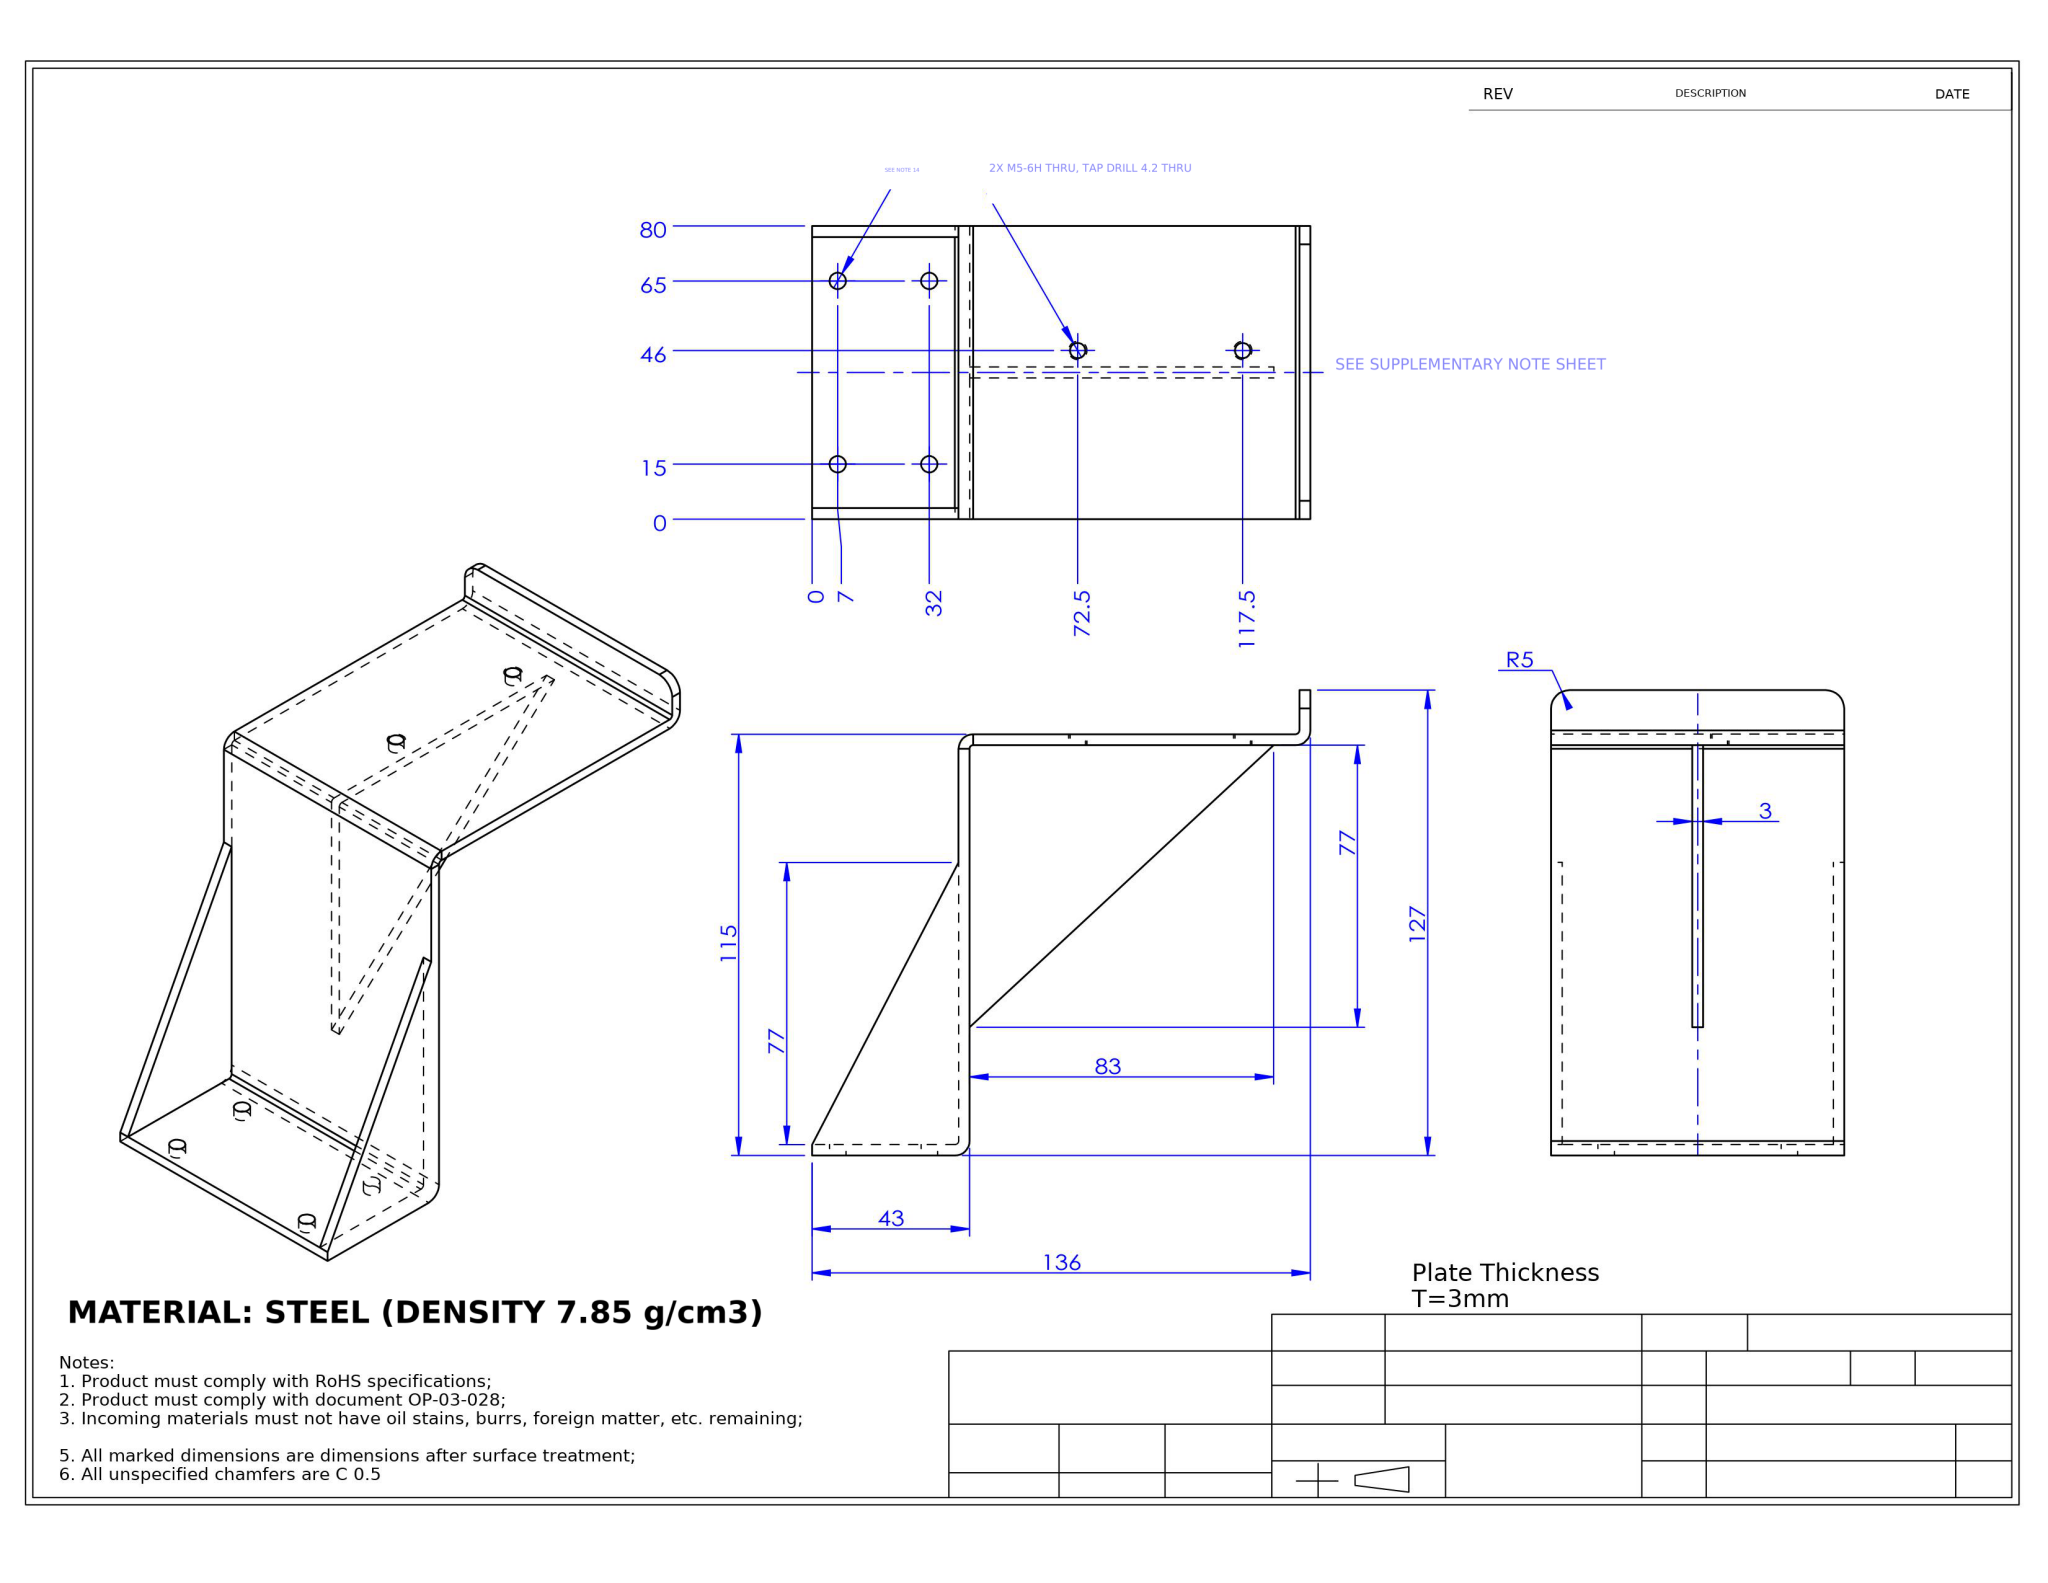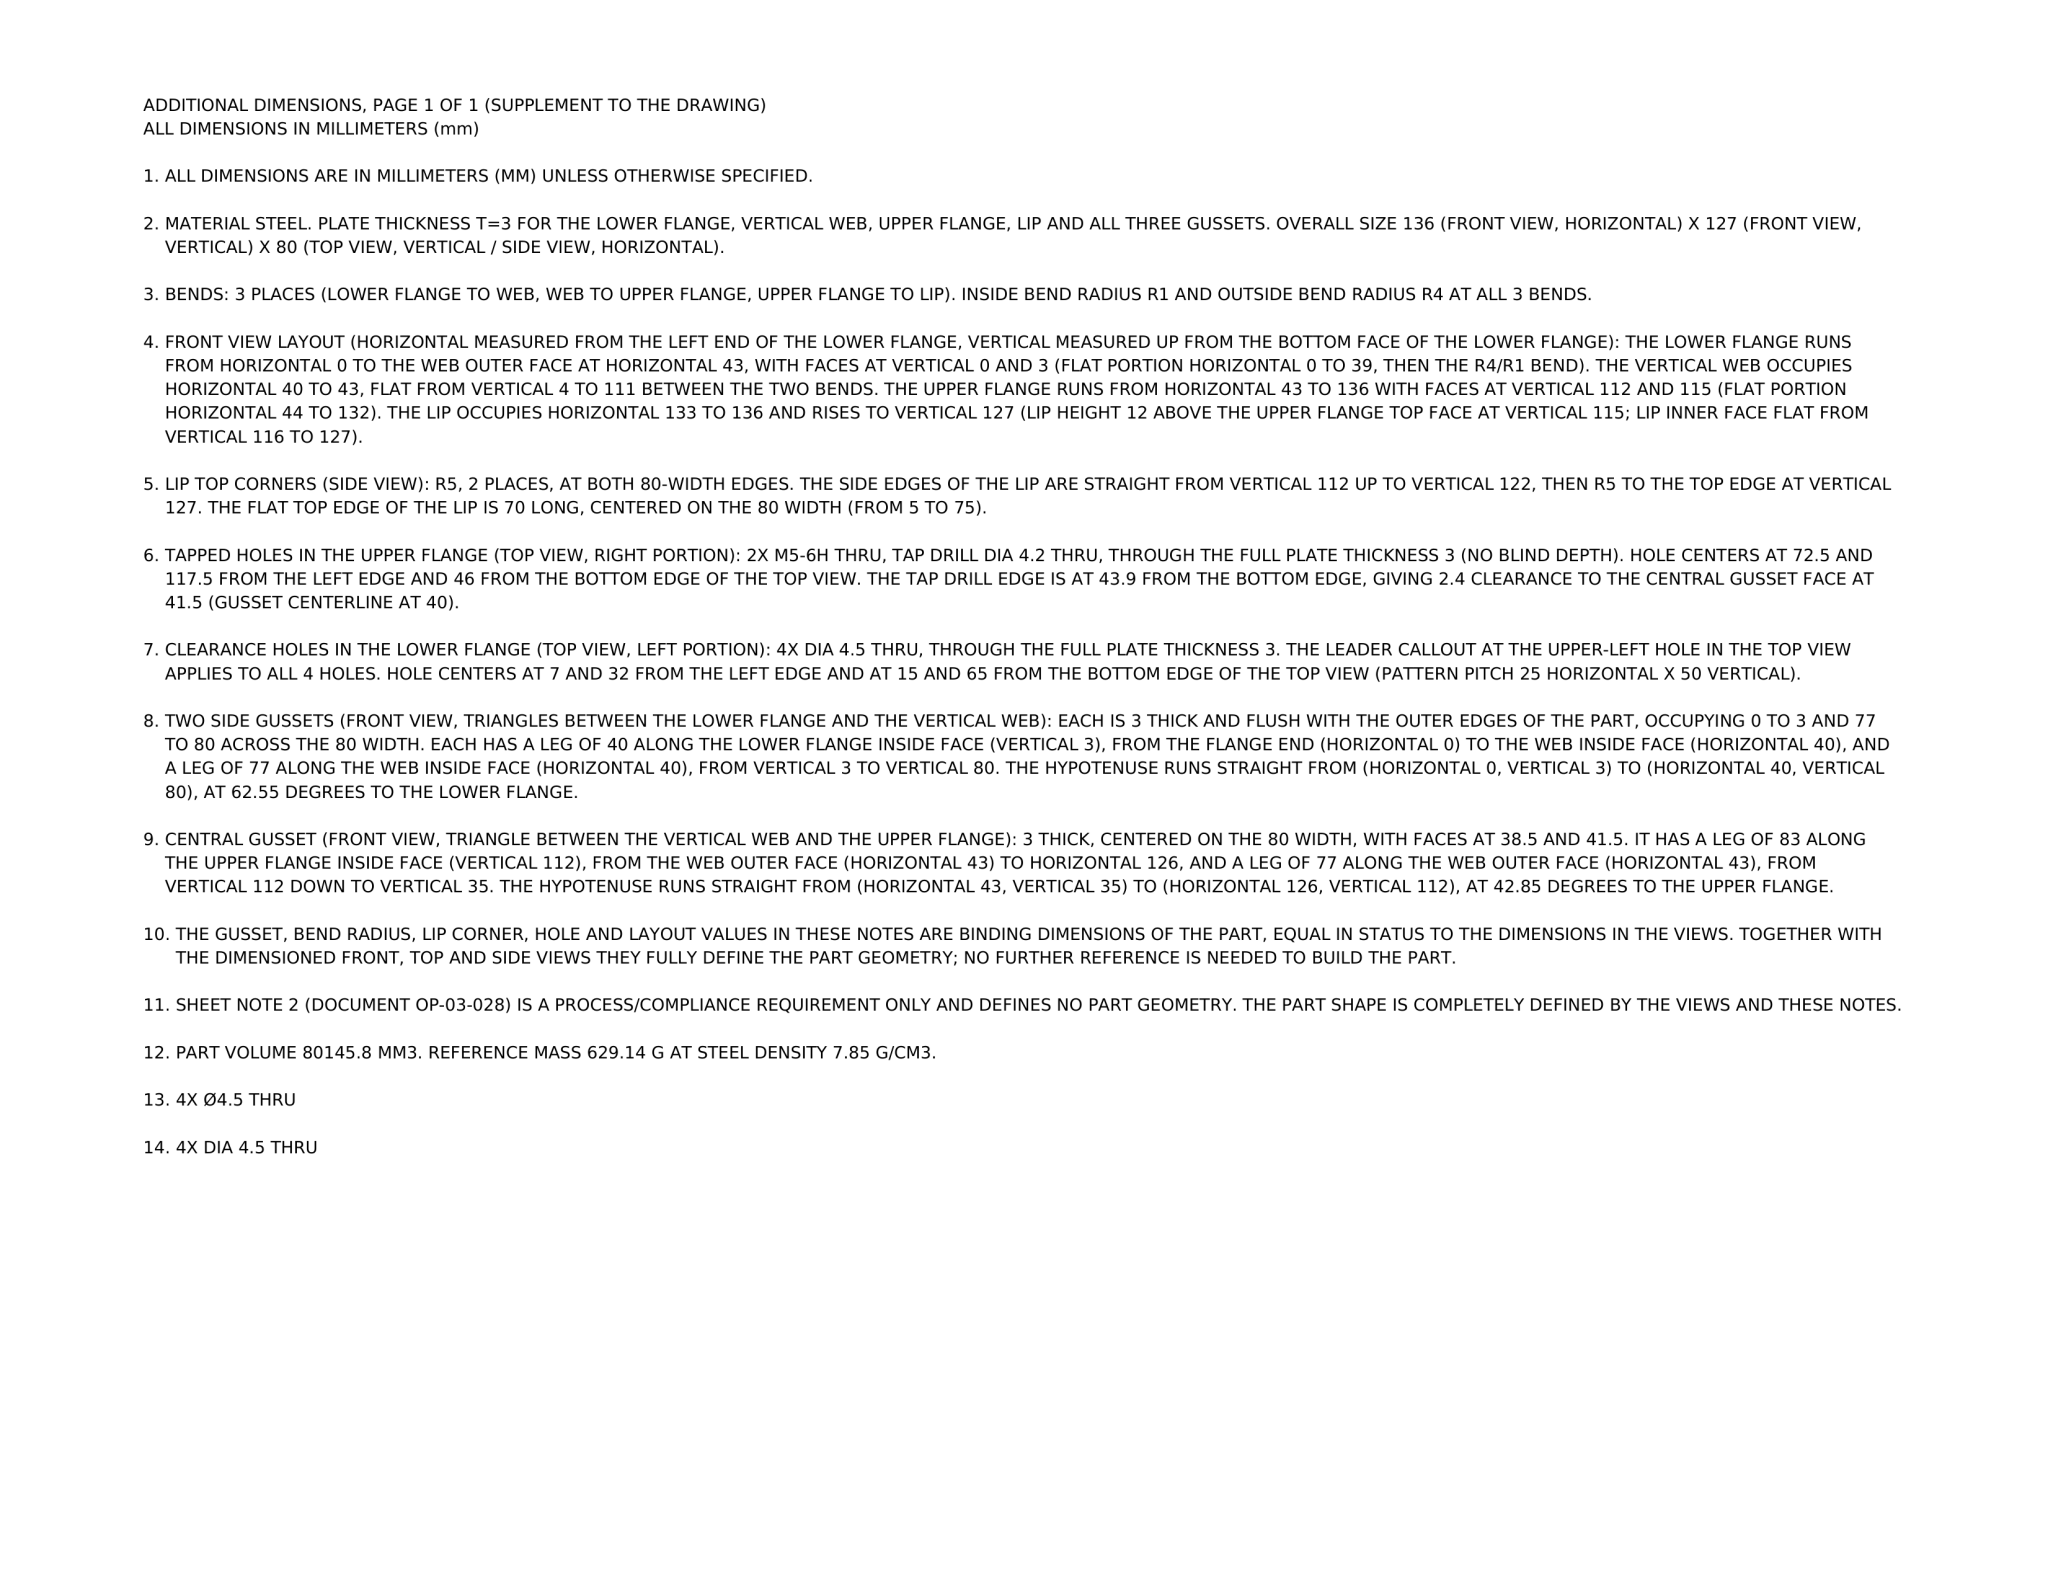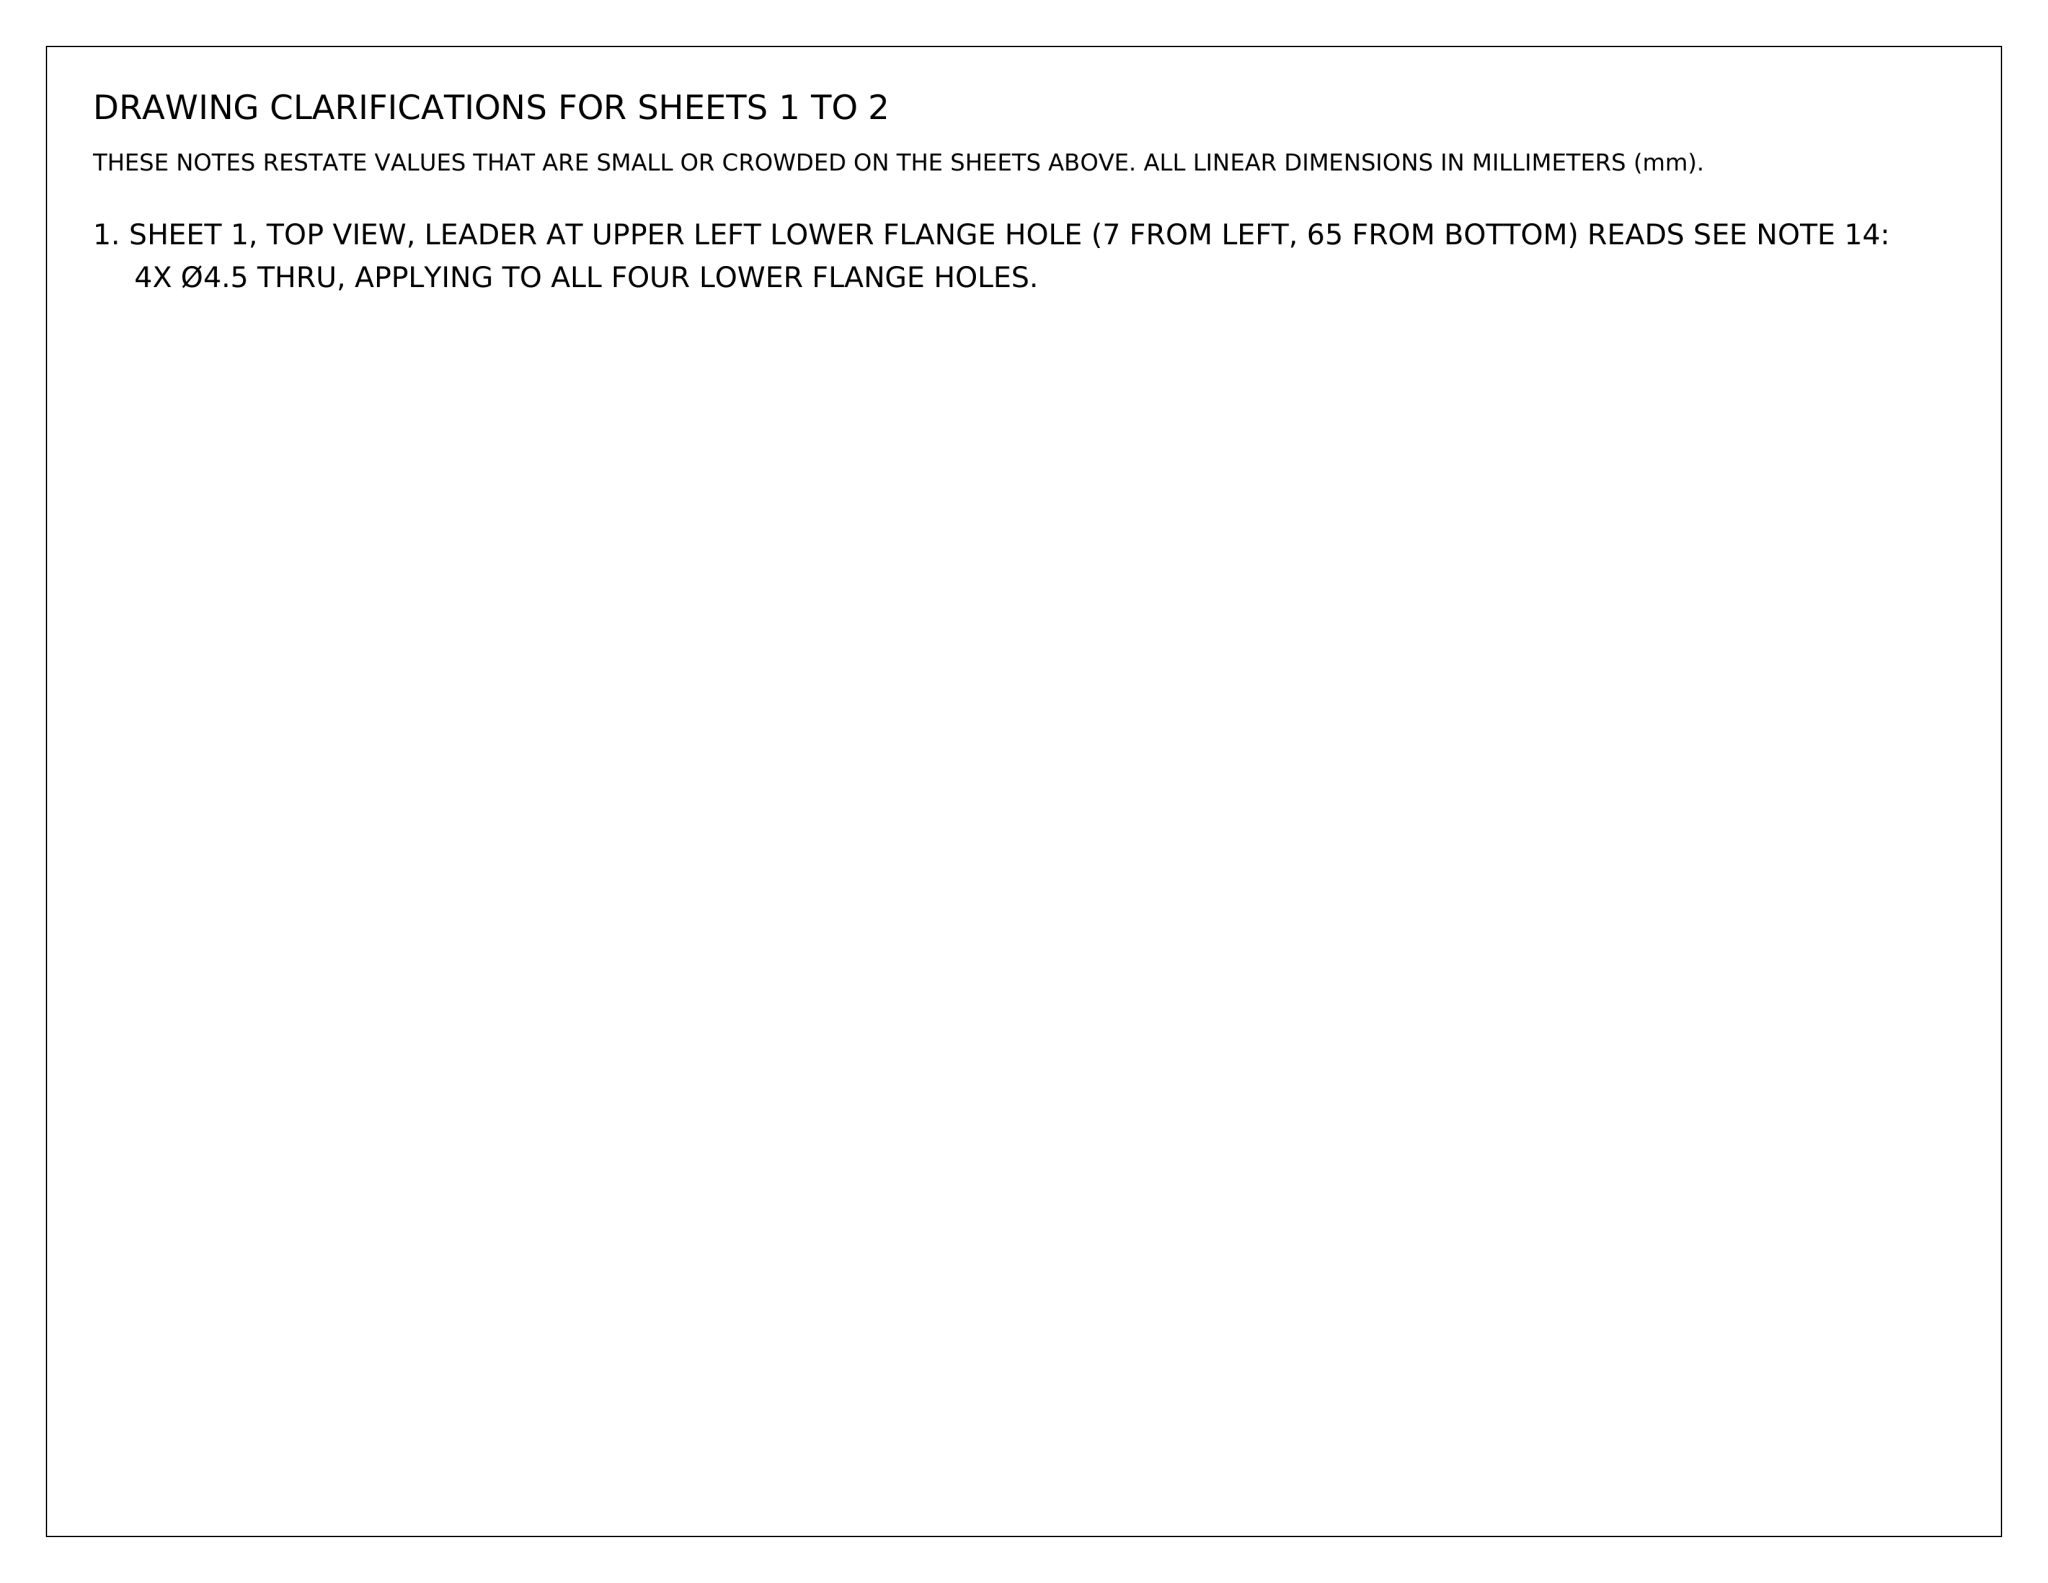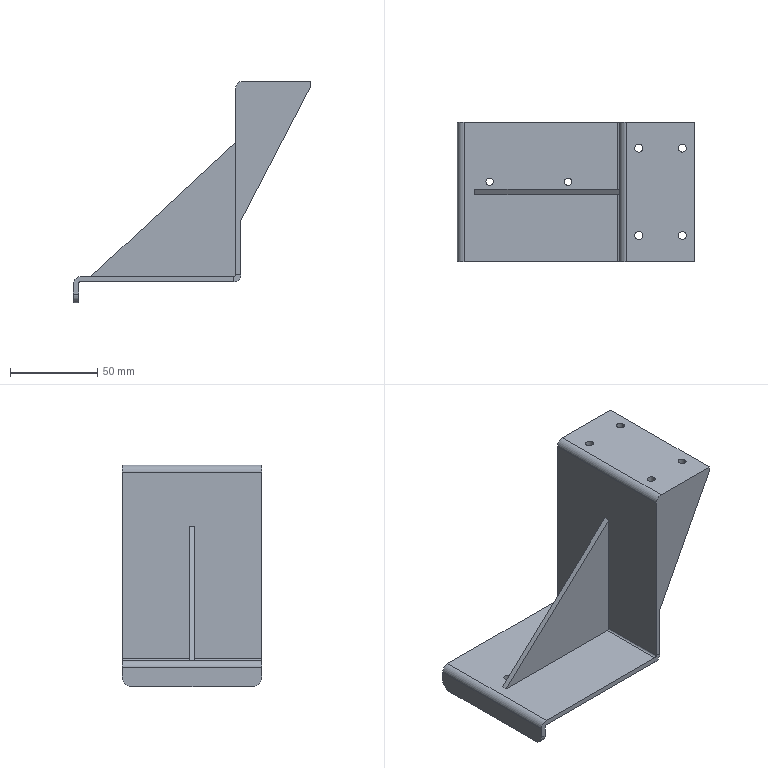Part | NX | mm | 1 solid | 44 faces | box 136 x 80 x 127 mm | volume 80146 mm3 | plane 23 | cylinder 21 | commonest cylinder face diameters 4.5 x8 4.2 x4 2 x4 8 x3 10 x2